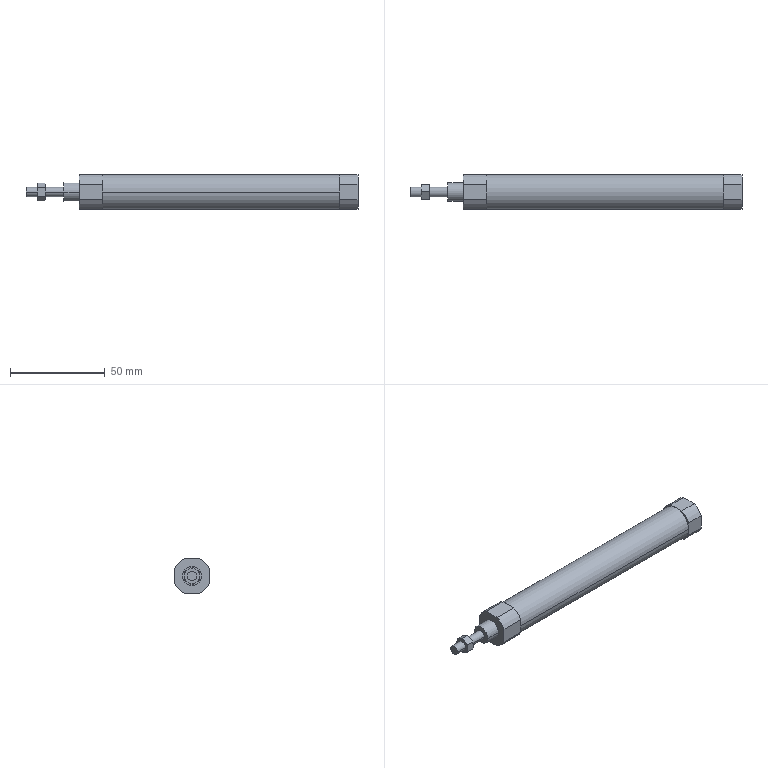Component | SolidWorks | CDJ2BSeries-1 | 1 solid | 64 faces | box 175 x 18.3 x 18.3 mm | volume 40358 mm3 | plane 30 | cylinder 20 | cone 14 | commonest cylinder face diameters 5 x8 20 x8 18.3 x2 10 x2